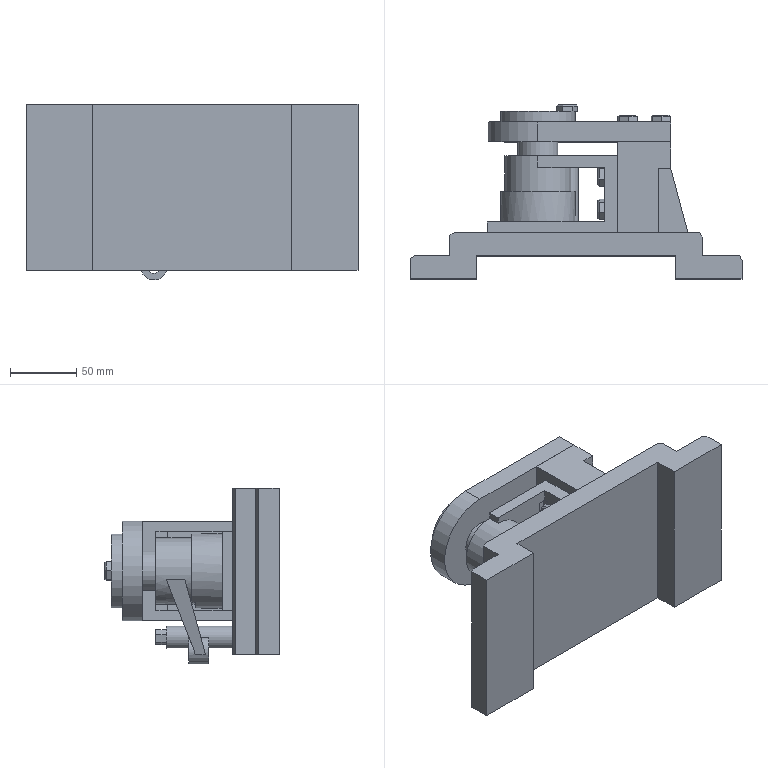Assembly | NX | mm | 15 component files | 15 solids | 276 faces | box 250 x 131.3 x 132.5 mm | volume 1237791 mm3 | plane 231 | cylinder 41 | cone 4 | commonest cylinder face diameters 10 x28 50 x3 30 x3 12 x2 56 x2 20 x1 75 x1 17 x1
Bill of materials:
unnamed part 1 | 1 |  | Flat plate of constant thickness with one end fully rounded and the other end square. It has a large through-hole centred on the rounded end, a small hole next to it, and four small holes in a rectangular 2x2 pattern near the square end.
unnamed part 2 | 9 |  | Fastener-like solid with a hexagonal head and a plain cylindrical shank. The head has chamfered corners on its outer face. The shank is shorter than about three head widths and has a flat end.
unnamed part 3 | 1 |  | Prismatic part with a constant cross-section along its length, shaped like an extrusion. The profile has a thin base web with stepped-down feet at both ends and a raised upright near one end with one tapered side. A small hooked or notched feature sits at the top of the upright, and shallow grooves or lands run along the length.
unnamed part 4 | 1 |  | Lever or crank-arm shape. A large hollow cylindrical boss is joined by a tapered web to a much smaller hollow cylindrical boss. The small boss is offset along the axis from the large boss, and the web runs at an angle between them.
unnamed part 5 | 1 |  | Stepped shaft with a larger-diameter cylindrical middle section. One end has a smaller round journal. The other end has a reduced stub with flat faces, apparently square or rectangular in section.
unnamed part 6 | 1 |  | Block-like bracket with a C-shaped side profile: a base plate, one vertical end wall, and a top flange that reaches only partway back over the base. The end wall has four through-holes in a 2x2 pattern. A short solid cylindrical boss or disc sits on the base under the open part of the top.
unnamed part 7 | 1 |  | Flanged pin: a plain cylindrical shank with a thin, larger-diameter circular flange at one end. The flange has one small through-hole placed off-centre near its rim.
Mates:
1. fix | jig_body 1 component
2. touch align | drill_bush_acc 1 face | jig_body 1 face
3. concentric | drill_bush_acc 1 edge | jig_body 1 edge
4. concentric | workpiece 1 edge | drill_bush_acc 1 edge
5. concentric | stop_pin 1 edge | jig_body 1 edge
6. concentric | mid_cyl_loc_pin 1 edge | drill_jig_bush 1 edge
7. align lock | mid_cyl_loc_pin 1 face | drill_jig_bush 1 face
8. concentric | loc_pin 2 edge | drill_jig_bush 1 edge
9. concentric | loc_pin 1 edge | drill_jig_bush 1 edge
10. concentric | loc_pin 8 edge | drill_jig_bush 1 edge
11. concentric | loc_pin 7 edge | drill_jig_bush 1 edge
12. concentric | loc_pin 6 edge | mid_cyl_loc_pin 1 edge
13. concentric | loc_pin 3 edge | drill_bush_acc 1 edge
14. concentric | loc_pin 4 edge | drill_bush_acc 1 edge
15. concentric | loc_pin 5 edge | drill_bush_acc 1 edge
16. concentric | loc_pin 9 edge | drill_bush_acc 1 edge